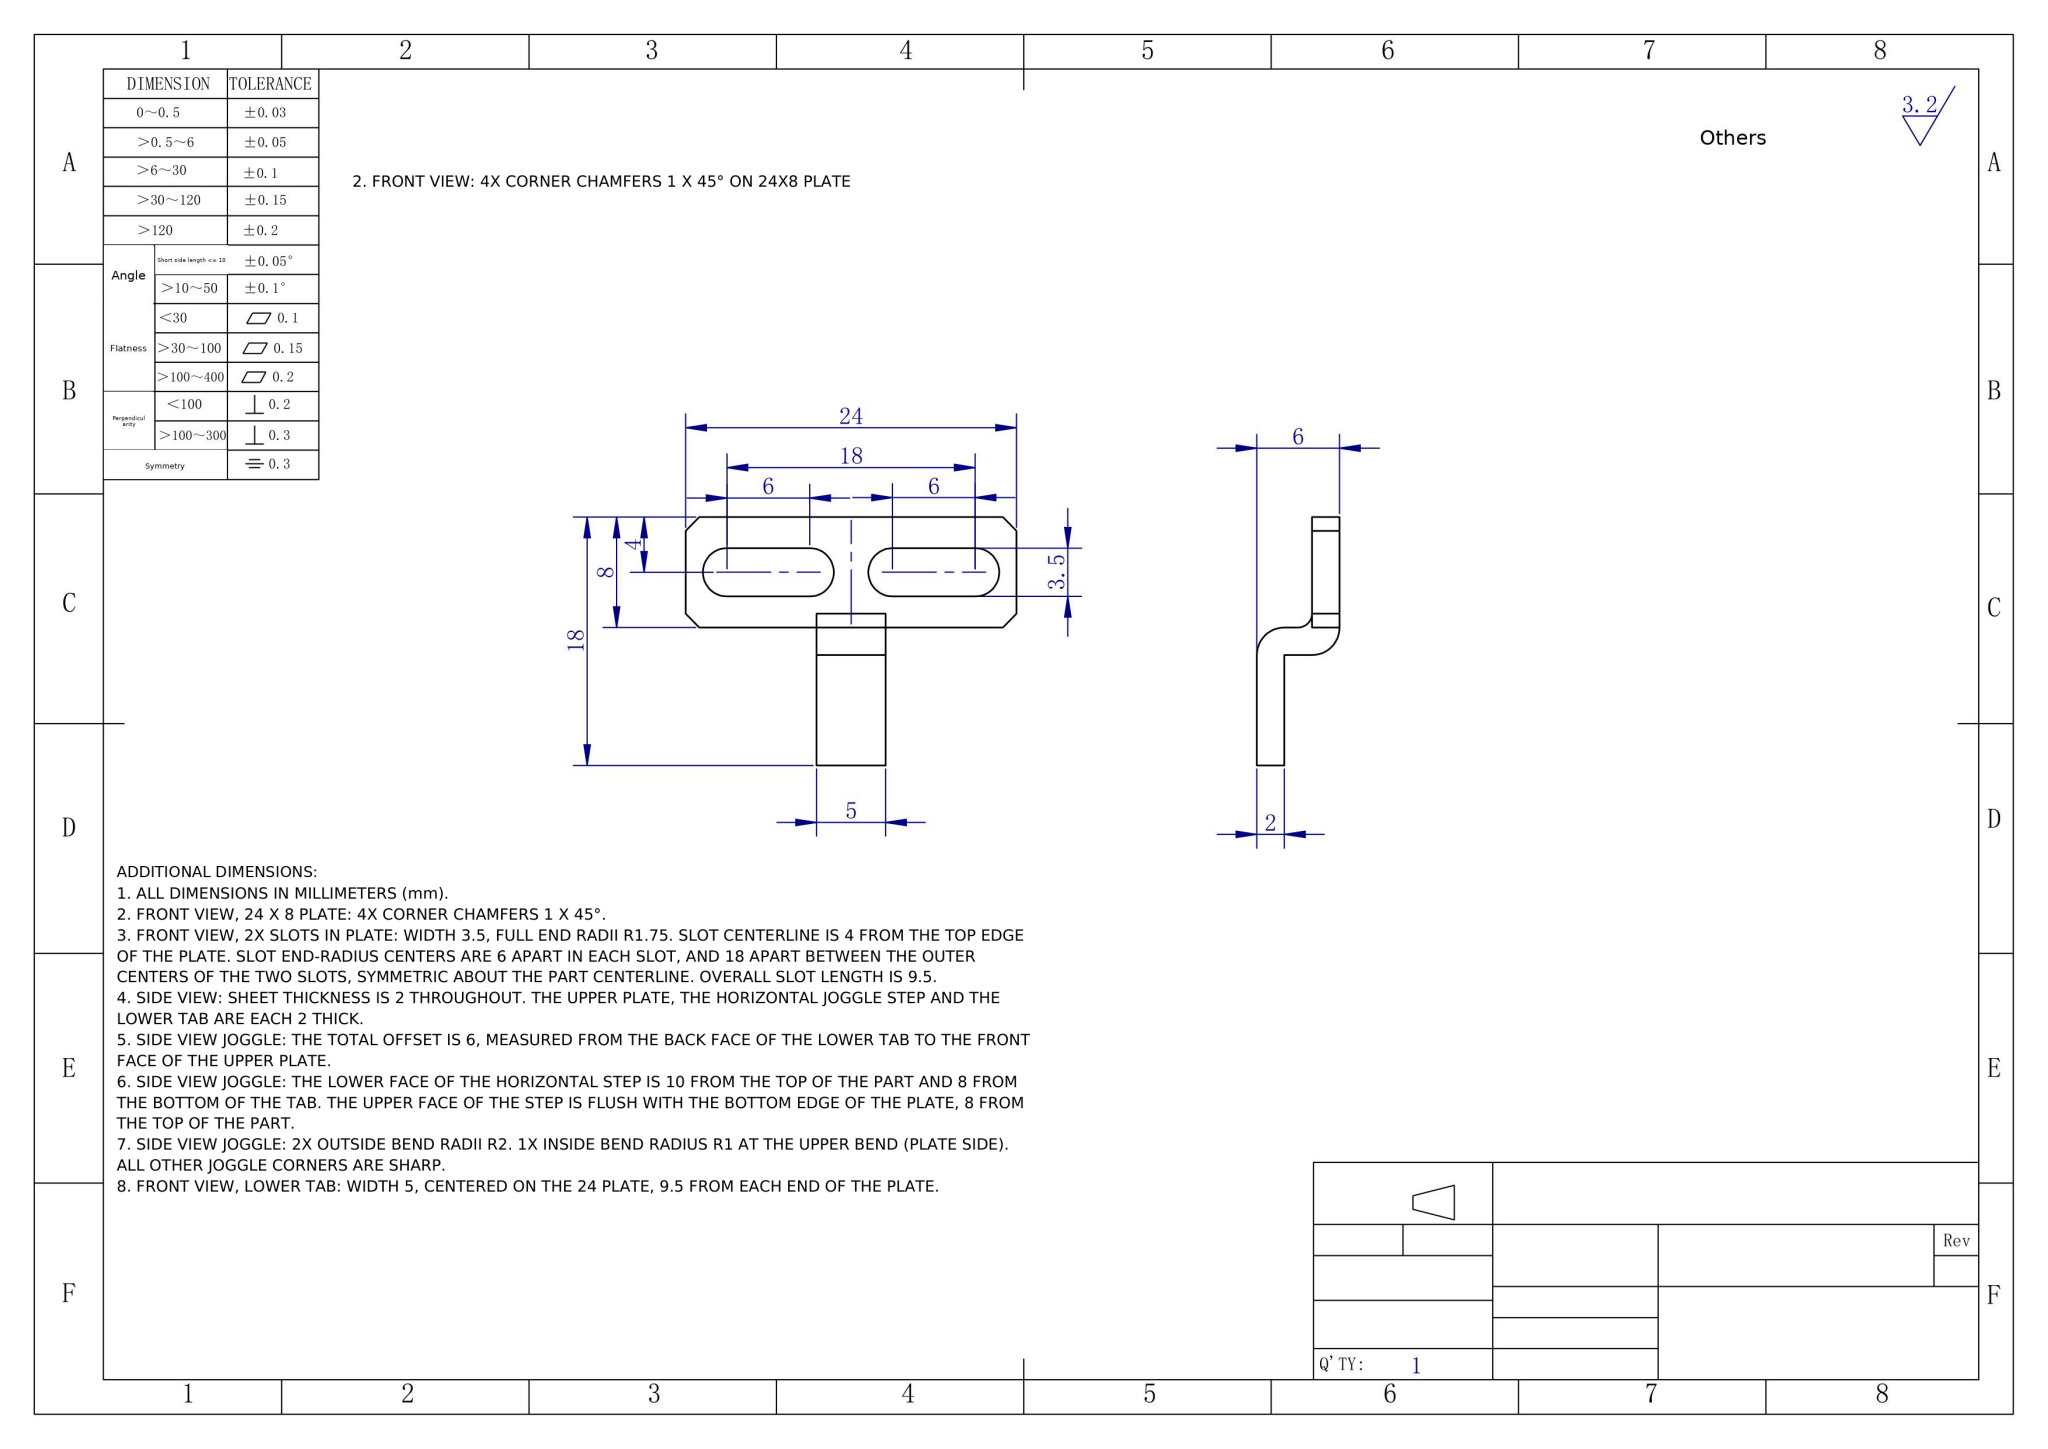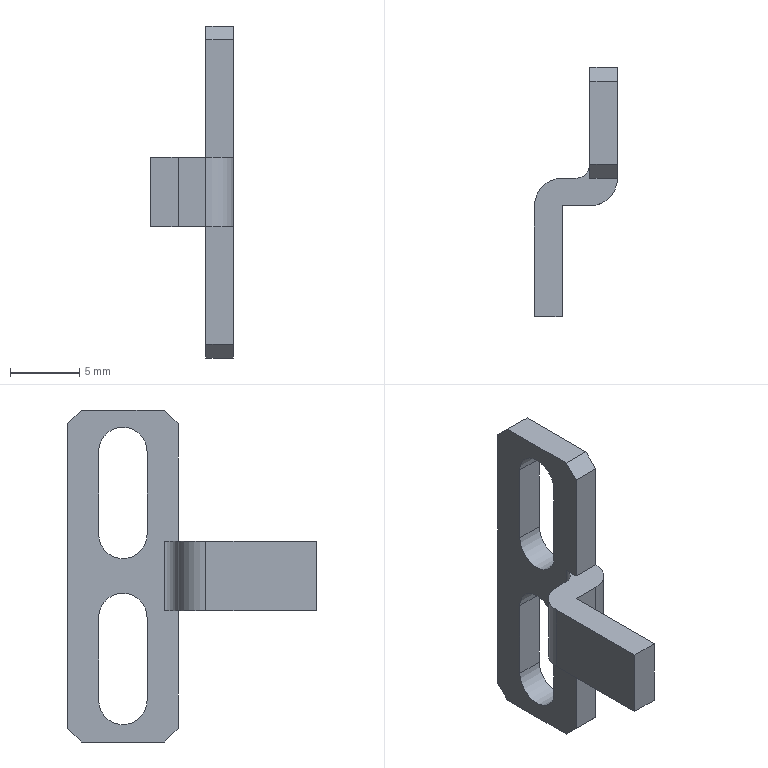Part | NX | mm | 1 solid | 31 faces | box 6 x 18 x 24 mm | volume 390 mm3 | plane 22 | cylinder 9 | commonest cylinder face diameters 3.5 x6 4 x2 2 x1
STEP:
#1=COLOUR_RGB('',0.7529,0.7529,0.7529);
#2=FILL_AREA_STYLE_COLOUR('',#1);
#3=FILL_AREA_STYLE('',(#2));
#4=SURFACE_STYLE_FILL_AREA(#3);
#5=SURFACE_SIDE_STYLE('',(#4));
#6=SURFACE_STYLE_USAGE(.BOTH.,#5);
#7=PRESENTATION_STYLE_ASSIGNMENT((#6));
#8=CARTESIAN_POINT('',(6.,4.,22.75));
#9=VERTEX_POINT('',#8);
#10=CARTESIAN_POINT('',(6.,5.75,21.));
#11=VERTEX_POINT('',#10);
#12=CARTESIAN_POINT('',(6.,4.,21.));
#13=DIRECTION('',(-1.,0.,0.));
#14=DIRECTION('',(0.,0.,1.));
#15=AXIS2_PLACEMENT_3D('',#12,#13,#14);
#16=CIRCLE('',#15,1.75);
#17=EDGE_CURVE('',#9,#11,#16,.T.);
#18=ORIENTED_EDGE('',*,*,#17,.F.);
#19=CARTESIAN_POINT('',(4.,4.,22.75));
#20=VERTEX_POINT('',#19);
#21=CARTESIAN_POINT('',(6.,4.,22.75));
#22=DIRECTION('',(-1.,0.,0.));
#23=VECTOR('',#22,1000.);
#24=LINE('',#21,#23);
#25=EDGE_CURVE('',#9,#20,#24,.T.);
#26=ORIENTED_EDGE('',*,*,#25,.T.);
#27=CARTESIAN_POINT('',(4.,5.75,21.));
#28=VERTEX_POINT('',#27);
#29=CARTESIAN_POINT('',(4.,4.,21.));
#30=DIRECTION('',(-1.,0.,0.));
#31=DIRECTION('',(0.,0.,1.));
#32=AXIS2_PLACEMENT_3D('',#29,#30,#31);
#33=CIRCLE('',#32,1.75);
#34=EDGE_CURVE('',#20,#28,#33,.T.);
#35=ORIENTED_EDGE('',*,*,#34,.T.);
#36=CARTESIAN_POINT('',(6.,5.75,21.));
#37=DIRECTION('',(-1.,0.,0.));
#38=VECTOR('',#37,1000.);
#39=LINE('',#36,#38);
#40=EDGE_CURVE('',#11,#28,#39,.T.);
#41=ORIENTED_EDGE('',*,*,#40,.F.);
#42=EDGE_LOOP('',(#18,#26,#35,#41));
#43=FACE_OUTER_BOUND('',#42,.T.);
#44=CARTESIAN_POINT('',(6.,4.,21.));
#45=DIRECTION('',(-1.,0.,0.));
#46=DIRECTION('',(0.,0.,1.));
#47=AXIS2_PLACEMENT_3D('',#44,#45,#46);
#48=CYLINDRICAL_SURFACE('',#47,1.75);
#49=ADVANCED_FACE('',(#43),#48,.F.);
#50=CARTESIAN_POINT('',(6.,4.,10.75));
#51=VERTEX_POINT('',#50);
#52=CARTESIAN_POINT('',(6.,5.75,9.));
#53=VERTEX_POINT('',#52);
#54=CARTESIAN_POINT('',(6.,4.,9.));
#55=DIRECTION('',(-1.,0.,0.));
#56=DIRECTION('',(0.,0.,1.));
#57=AXIS2_PLACEMENT_3D('',#54,#55,#56);
#58=CIRCLE('',#57,1.75);
#59=EDGE_CURVE('',#51,#53,#58,.T.);
#60=ORIENTED_EDGE('',*,*,#59,.F.);
#61=CARTESIAN_POINT('',(4.,4.,10.75));
#62=VERTEX_POINT('',#61);
#63=CARTESIAN_POINT('',(6.,4.,10.75));
#64=DIRECTION('',(-1.,0.,0.));
#65=VECTOR('',#64,1000.);
#66=LINE('',#63,#65);
#67=EDGE_CURVE('',#51,#62,#66,.T.);
#68=ORIENTED_EDGE('',*,*,#67,.T.);
#69=CARTESIAN_POINT('',(4.,5.75,9.));
#70=VERTEX_POINT('',#69);
#71=CARTESIAN_POINT('',(4.,4.,9.));
#72=DIRECTION('',(-1.,0.,0.));
#73=DIRECTION('',(0.,0.,1.));
#74=AXIS2_PLACEMENT_3D('',#71,#72,#73);
#75=CIRCLE('',#74,1.75);
#76=EDGE_CURVE('',#62,#70,#75,.T.);
#77=ORIENTED_EDGE('',*,*,#76,.T.);
#78=CARTESIAN_POINT('',(6.,5.75,9.));
#79=DIRECTION('',(-1.,0.,0.));
#80=VECTOR('',#79,1000.);
#81=LINE('',#78,#80);
#82=EDGE_CURVE('',#53,#70,#81,.T.);
#83=ORIENTED_EDGE('',*,*,#82,.F.);
#84=EDGE_LOOP('',(#60,#68,#77,#83));
#85=FACE_OUTER_BOUND('',#84,.T.);
#86=CARTESIAN_POINT('',(6.,4.,9.));
#87=DIRECTION('',(-1.,0.,0.));
#88=DIRECTION('',(0.,0.,1.));
#89=AXIS2_PLACEMENT_3D('',#86,#87,#88);
#90=CYLINDRICAL_SURFACE('',#89,1.75);
#91=ADVANCED_FACE('',(#85),#90,.F.);
#92=CARTESIAN_POINT('',(4.,1.,24.));
#93=VERTEX_POINT('',#92);
#94=CARTESIAN_POINT('',(4.,7.,24.));
#95=VERTEX_POINT('',#94);
#96=CARTESIAN_POINT('',(4.,0.,24.));
#97=DIRECTION('',(0.,1.,0.));
#98=VECTOR('',#97,1000.);
#99=LINE('',#96,#98);
#100=EDGE_CURVE('',#93,#95,#99,.T.);
#101=ORIENTED_EDGE('',*,*,#100,.F.);
#102=CARTESIAN_POINT('',(6.,1.,24.));
#103=VERTEX_POINT('',#102);
#104=CARTESIAN_POINT('',(0.,1.,24.));
#105=DIRECTION('',(1.,0.,0.));
#106=VECTOR('',#105,1000.);
#107=LINE('',#104,#106);
#108=EDGE_CURVE('',#93,#103,#107,.T.);
#109=ORIENTED_EDGE('',*,*,#108,.T.);
#110=CARTESIAN_POINT('',(6.,7.,24.));
#111=VERTEX_POINT('',#110);
#112=CARTESIAN_POINT('',(6.,0.,24.));
#113=DIRECTION('',(0.,1.,0.));
#114=VECTOR('',#113,1000.);
#115=LINE('',#112,#114);
#116=EDGE_CURVE('',#103,#111,#115,.T.);
#117=ORIENTED_EDGE('',*,*,#116,.T.);
#118=CARTESIAN_POINT('',(4.,7.,24.));
#119=DIRECTION('',(-1.,0.,0.));
#120=VECTOR('',#119,1000.);
#121=LINE('',#118,#120);
#122=EDGE_CURVE('',#111,#95,#121,.T.);
#123=ORIENTED_EDGE('',*,*,#122,.T.);
#124=EDGE_LOOP('',(#101,#109,#117,#123));
#125=FACE_OUTER_BOUND('',#124,.T.);
#126=CARTESIAN_POINT('',(0.,0.,24.));
#127=DIRECTION('',(0.,0.,-1.));
#128=DIRECTION('',(-1.,0.,0.));
#129=AXIS2_PLACEMENT_3D('',#126,#127,#128);
#130=PLANE('',#129);
#131=ADVANCED_FACE('',(#125),#130,.F.);
#132=CARTESIAN_POINT('',(6.,5.75,15.));
#133=VERTEX_POINT('',#132);
#134=CARTESIAN_POINT('',(6.,5.75,15.));
#135=DIRECTION('',(0.,-0.,-1.));
#136=VECTOR('',#135,1000.);
#137=LINE('',#134,#136);
#138=EDGE_CURVE('',#11,#133,#137,.T.);
#139=ORIENTED_EDGE('',*,*,#138,.T.);
#140=CARTESIAN_POINT('',(6.,2.25,15.));
#141=VERTEX_POINT('',#140);
#142=CARTESIAN_POINT('',(6.,4.,15.));
#143=DIRECTION('',(-1.,0.,0.));
#144=DIRECTION('',(0.,0.,1.));
#145=AXIS2_PLACEMENT_3D('',#142,#143,#144);
#146=CIRCLE('',#145,1.75);
#147=EDGE_CURVE('',#133,#141,#146,.T.);
#148=ORIENTED_EDGE('',*,*,#147,.T.);
#149=CARTESIAN_POINT('',(6.,2.25,21.));
#150=VERTEX_POINT('',#149);
#151=CARTESIAN_POINT('',(6.,2.25,15.));
#152=DIRECTION('',(0.,0.,1.));
#153=VECTOR('',#152,1000.);
#154=LINE('',#151,#153);
#155=EDGE_CURVE('',#141,#150,#154,.T.);
#156=ORIENTED_EDGE('',*,*,#155,.T.);
#157=CARTESIAN_POINT('',(6.,4.,21.));
#158=DIRECTION('',(-1.,0.,0.));
#159=DIRECTION('',(0.,0.,1.));
#160=AXIS2_PLACEMENT_3D('',#157,#158,#159);
#161=CIRCLE('',#160,1.75);
#162=EDGE_CURVE('',#150,#9,#161,.T.);
#163=ORIENTED_EDGE('',*,*,#162,.T.);
#164=ORIENTED_EDGE('',*,*,#17,.T.);
#165=EDGE_LOOP('',(#139,#148,#156,#163,#164));
#166=FACE_BOUND('',#165,.T.);
#167=CARTESIAN_POINT('',(6.,5.75,3.));
#168=VERTEX_POINT('',#167);
#169=CARTESIAN_POINT('',(6.,5.75,3.));
#170=DIRECTION('',(0.,-0.,-1.));
#171=VECTOR('',#170,1000.);
#172=LINE('',#169,#171);
#173=EDGE_CURVE('',#53,#168,#172,.T.);
#174=ORIENTED_EDGE('',*,*,#173,.T.);
#175=CARTESIAN_POINT('',(6.,2.25,3.));
#176=VERTEX_POINT('',#175);
#177=CARTESIAN_POINT('',(6.,4.,3.));
#178=DIRECTION('',(-1.,0.,0.));
#179=DIRECTION('',(0.,0.,1.));
#180=AXIS2_PLACEMENT_3D('',#177,#178,#179);
#181=CIRCLE('',#180,1.75);
#182=EDGE_CURVE('',#168,#176,#181,.T.);
#183=ORIENTED_EDGE('',*,*,#182,.T.);
#184=CARTESIAN_POINT('',(6.,2.25,9.));
#185=VERTEX_POINT('',#184);
#186=CARTESIAN_POINT('',(6.,2.25,3.));
#187=DIRECTION('',(0.,0.,1.));
#188=VECTOR('',#187,1000.);
#189=LINE('',#186,#188);
#190=EDGE_CURVE('',#176,#185,#189,.T.);
#191=ORIENTED_EDGE('',*,*,#190,.T.);
#192=CARTESIAN_POINT('',(6.,4.,9.));
#193=DIRECTION('',(-1.,0.,0.));
#194=DIRECTION('',(0.,0.,1.));
#195=AXIS2_PLACEMENT_3D('',#192,#193,#194);
#196=CIRCLE('',#195,1.75);
#197=EDGE_CURVE('',#185,#51,#196,.T.);
#198=ORIENTED_EDGE('',*,*,#197,.T.);
#199=ORIENTED_EDGE('',*,*,#59,.T.);
#200=EDGE_LOOP('',(#174,#183,#191,#198,#199));
#201=FACE_BOUND('',#200,.T.);
#202=ORIENTED_EDGE('',*,*,#116,.F.);
#203=CARTESIAN_POINT('',(6.,0.,23.));
#204=VERTEX_POINT('',#203);
#205=CARTESIAN_POINT('',(6.,1.,24.));
#206=DIRECTION('',(0.,-0.7071,-0.7071));
#207=VECTOR('',#206,1000.);
#208=LINE('',#205,#207);
#209=EDGE_CURVE('',#103,#204,#208,.T.);
#210=ORIENTED_EDGE('',*,*,#209,.T.);
#211=CARTESIAN_POINT('',(6.,0.,14.5));
#212=VERTEX_POINT('',#211);
#213=CARTESIAN_POINT('',(6.,0.,24.));
#214=DIRECTION('',(0.,0.,-1.));
#215=VECTOR('',#214,1000.);
#216=LINE('',#213,#215);
#217=EDGE_CURVE('',#204,#212,#216,.T.);
#218=ORIENTED_EDGE('',*,*,#217,.T.);
#219=CARTESIAN_POINT('',(6.,0.,9.5));
#220=VERTEX_POINT('',#219);
#221=CARTESIAN_POINT('',(6.,0.,24.));
#222=DIRECTION('',(0.,0.,-1.));
#223=VECTOR('',#222,1000.);
#224=LINE('',#221,#223);
#225=EDGE_CURVE('',#212,#220,#224,.T.);
#226=ORIENTED_EDGE('',*,*,#225,.T.);
#227=CARTESIAN_POINT('',(6.,-0.,1.));
#228=VERTEX_POINT('',#227);
#229=CARTESIAN_POINT('',(6.,0.,24.));
#230=DIRECTION('',(0.,0.,-1.));
#231=VECTOR('',#230,1000.);
#232=LINE('',#229,#231);
#233=EDGE_CURVE('',#220,#228,#232,.T.);
#234=ORIENTED_EDGE('',*,*,#233,.T.);
#235=CARTESIAN_POINT('',(6.,1.,0.));
#236=VERTEX_POINT('',#235);
#237=CARTESIAN_POINT('',(6.,0.,1.));
#238=DIRECTION('',(0.,0.7071,-0.7071));
#239=VECTOR('',#238,1000.);
#240=LINE('',#237,#239);
#241=EDGE_CURVE('',#228,#236,#240,.T.);
#242=ORIENTED_EDGE('',*,*,#241,.T.);
#243=CARTESIAN_POINT('',(6.,7.,0.));
#244=VERTEX_POINT('',#243);
#245=CARTESIAN_POINT('',(6.,0.,0.));
#246=DIRECTION('',(0.,1.,0.));
#247=VECTOR('',#246,1000.);
#248=LINE('',#245,#247);
#249=EDGE_CURVE('',#236,#244,#248,.T.);
#250=ORIENTED_EDGE('',*,*,#249,.T.);
#251=CARTESIAN_POINT('',(6.,8.,1.));
#252=VERTEX_POINT('',#251);
#253=CARTESIAN_POINT('',(6.,7.,0.));
#254=DIRECTION('',(0.,0.7071,0.7071));
#255=VECTOR('',#254,1000.);
#256=LINE('',#253,#255);
#257=EDGE_CURVE('',#244,#252,#256,.T.);
#258=ORIENTED_EDGE('',*,*,#257,.T.);
#259=CARTESIAN_POINT('',(6.,8.,23.));
#260=VERTEX_POINT('',#259);
#261=CARTESIAN_POINT('',(6.,8.,24.));
#262=DIRECTION('',(0.,0.,-1.));
#263=VECTOR('',#262,1000.);
#264=LINE('',#261,#263);
#265=EDGE_CURVE('',#260,#252,#264,.T.);
#266=ORIENTED_EDGE('',*,*,#265,.F.);
#267=CARTESIAN_POINT('',(6.,8.,23.));
#268=DIRECTION('',(0.,-0.7071,0.7071));
#269=VECTOR('',#268,1000.);
#270=LINE('',#267,#269);
#271=EDGE_CURVE('',#260,#111,#270,.T.);
#272=ORIENTED_EDGE('',*,*,#271,.T.);
#273=EDGE_LOOP('',(#202,#210,#218,#226,#234,#242,#250,#258,#266,#272));
#274=FACE_OUTER_BOUND('',#273,.T.);
#275=CARTESIAN_POINT('',(6.,0.,24.));
#276=DIRECTION('',(-1.,0.,0.));
#277=DIRECTION('',(0.,0.,1.));
#278=AXIS2_PLACEMENT_3D('',#275,#276,#277);
#279=PLANE('',#278);
#280=ADVANCED_FACE('',(#166,#201,#274),#279,.F.);
#281=CARTESIAN_POINT('',(4.,8.,23.));
#282=VERTEX_POINT('',#281);
#283=CARTESIAN_POINT('',(4.,8.,1.));
#284=VERTEX_POINT('',#283);
#285=CARTESIAN_POINT('',(4.,8.,24.));
#286=DIRECTION('',(0.,0.,-1.));
#287=VECTOR('',#286,1000.);
#288=LINE('',#285,#287);
#289=EDGE_CURVE('',#282,#284,#288,.T.);
#290=ORIENTED_EDGE('',*,*,#289,.F.);
#291=CARTESIAN_POINT('',(6.,8.,23.));
#292=DIRECTION('',(1.,0.,0.));
#293=VECTOR('',#292,1000.);
#294=LINE('',#291,#293);
#295=EDGE_CURVE('',#282,#260,#294,.T.);
#296=ORIENTED_EDGE('',*,*,#295,.T.);
#297=ORIENTED_EDGE('',*,*,#265,.T.);
#298=CARTESIAN_POINT('',(4.,8.,1.));
#299=DIRECTION('',(-1.,0.,0.));
#300=VECTOR('',#299,1000.);
#301=LINE('',#298,#300);
#302=EDGE_CURVE('',#252,#284,#301,.T.);
#303=ORIENTED_EDGE('',*,*,#302,.T.);
#304=EDGE_LOOP('',(#290,#296,#297,#303));
#305=FACE_OUTER_BOUND('',#304,.T.);
#306=CARTESIAN_POINT('',(4.,8.,24.));
#307=DIRECTION('',(0.,1.,0.));
#308=DIRECTION('',(0.,0.,1.));
#309=AXIS2_PLACEMENT_3D('',#306,#307,#308);
#310=PLANE('',#309);
#311=ADVANCED_FACE('',(#305),#310,.T.);
#312=CARTESIAN_POINT('',(4.,5.75,15.));
#313=VERTEX_POINT('',#312);
#314=CARTESIAN_POINT('',(4.,2.25,15.));
#315=VERTEX_POINT('',#314);
#316=CARTESIAN_POINT('',(4.,4.,15.));
#317=DIRECTION('',(-1.,0.,0.));
#318=DIRECTION('',(0.,0.,1.));
#319=AXIS2_PLACEMENT_3D('',#316,#317,#318);
#320=CIRCLE('',#319,1.75);
#321=EDGE_CURVE('',#313,#315,#320,.T.);
#322=ORIENTED_EDGE('',*,*,#321,.F.);
#323=CARTESIAN_POINT('',(4.,5.75,15.));
#324=DIRECTION('',(0.,-0.,-1.));
#325=VECTOR('',#324,1000.);
#326=LINE('',#323,#325);
#327=EDGE_CURVE('',#28,#313,#326,.T.);
#328=ORIENTED_EDGE('',*,*,#327,.F.);
#329=ORIENTED_EDGE('',*,*,#34,.F.);
#330=CARTESIAN_POINT('',(4.,2.25,21.));
#331=VERTEX_POINT('',#330);
#332=CARTESIAN_POINT('',(4.,4.,21.));
#333=DIRECTION('',(-1.,0.,0.));
#334=DIRECTION('',(0.,0.,1.));
#335=AXIS2_PLACEMENT_3D('',#332,#333,#334);
#336=CIRCLE('',#335,1.75);
#337=EDGE_CURVE('',#331,#20,#336,.T.);
#338=ORIENTED_EDGE('',*,*,#337,.F.);
#339=CARTESIAN_POINT('',(4.,2.25,15.));
#340=DIRECTION('',(0.,0.,1.));
#341=VECTOR('',#340,1000.);
#342=LINE('',#339,#341);
#343=EDGE_CURVE('',#315,#331,#342,.T.);
#344=ORIENTED_EDGE('',*,*,#343,.F.);
#345=EDGE_LOOP('',(#322,#328,#329,#338,#344));
#346=FACE_BOUND('',#345,.T.);
#347=CARTESIAN_POINT('',(4.,5.75,3.));
#348=VERTEX_POINT('',#347);
#349=CARTESIAN_POINT('',(4.,2.25,3.));
#350=VERTEX_POINT('',#349);
#351=CARTESIAN_POINT('',(4.,4.,3.));
#352=DIRECTION('',(-1.,0.,0.));
#353=DIRECTION('',(0.,0.,1.));
#354=AXIS2_PLACEMENT_3D('',#351,#352,#353);
#355=CIRCLE('',#354,1.75);
#356=EDGE_CURVE('',#348,#350,#355,.T.);
#357=ORIENTED_EDGE('',*,*,#356,.F.);
#358=CARTESIAN_POINT('',(4.,5.75,3.));
#359=DIRECTION('',(0.,-0.,-1.));
#360=VECTOR('',#359,1000.);
#361=LINE('',#358,#360);
#362=EDGE_CURVE('',#70,#348,#361,.T.);
#363=ORIENTED_EDGE('',*,*,#362,.F.);
#364=ORIENTED_EDGE('',*,*,#76,.F.);
#365=CARTESIAN_POINT('',(4.,2.25,9.));
#366=VERTEX_POINT('',#365);
#367=CARTESIAN_POINT('',(4.,4.,9.));
#368=DIRECTION('',(-1.,0.,0.));
#369=DIRECTION('',(0.,0.,1.));
#370=AXIS2_PLACEMENT_3D('',#367,#368,#369);
#371=CIRCLE('',#370,1.75);
#372=EDGE_CURVE('',#366,#62,#371,.T.);
#373=ORIENTED_EDGE('',*,*,#372,.F.);
#374=CARTESIAN_POINT('',(4.,2.25,3.));
#375=DIRECTION('',(0.,0.,1.));
#376=VECTOR('',#375,1000.);
#377=LINE('',#374,#376);
#378=EDGE_CURVE('',#350,#366,#377,.T.);
#379=ORIENTED_EDGE('',*,*,#378,.F.);
#380=EDGE_LOOP('',(#357,#363,#364,#373,#379));
#381=FACE_BOUND('',#380,.T.);
#382=CARTESIAN_POINT('',(4.,0.,23.));
#383=VERTEX_POINT('',#382);
#384=CARTESIAN_POINT('',(4.,0.,14.5));
#385=VERTEX_POINT('',#384);
#386=CARTESIAN_POINT('',(4.,0.,24.));
#387=DIRECTION('',(0.,0.,-1.));
#388=VECTOR('',#387,1000.);
#389=LINE('',#386,#388);
#390=EDGE_CURVE('',#383,#385,#389,.T.);
#391=ORIENTED_EDGE('',*,*,#390,.F.);
#392=CARTESIAN_POINT('',(4.,0.5,23.5));
#393=DIRECTION('',(0.,0.7071,0.7071));
#394=VECTOR('',#393,1000.);
#395=LINE('',#392,#394);
#396=EDGE_CURVE('',#383,#93,#395,.T.);
#397=ORIENTED_EDGE('',*,*,#396,.T.);
#398=ORIENTED_EDGE('',*,*,#100,.T.);
#399=CARTESIAN_POINT('',(4.,3.5,27.5));
#400=DIRECTION('',(0.,0.7071,-0.7071));
#401=VECTOR('',#400,1000.);
#402=LINE('',#399,#401);
#403=EDGE_CURVE('',#95,#282,#402,.T.);
#404=ORIENTED_EDGE('',*,*,#403,.T.);
#405=ORIENTED_EDGE('',*,*,#289,.T.);
#406=CARTESIAN_POINT('',(4.,7.,0.));
#407=VERTEX_POINT('',#406);
#408=CARTESIAN_POINT('',(4.,15.5,8.5));
#409=DIRECTION('',(0.,-0.7071,-0.7071));
#410=VECTOR('',#409,1000.);
#411=LINE('',#408,#410);
#412=EDGE_CURVE('',#284,#407,#411,.T.);
#413=ORIENTED_EDGE('',*,*,#412,.T.);
#414=CARTESIAN_POINT('',(4.,1.,0.));
#415=VERTEX_POINT('',#414);
#416=CARTESIAN_POINT('',(4.,0.,0.));
#417=DIRECTION('',(0.,1.,0.));
#418=VECTOR('',#417,1000.);
#419=LINE('',#416,#418);
#420=EDGE_CURVE('',#415,#407,#419,.T.);
#421=ORIENTED_EDGE('',*,*,#420,.F.);
#422=CARTESIAN_POINT('',(4.,-0.,1.));
#423=VERTEX_POINT('',#422);
#424=CARTESIAN_POINT('',(4.,-11.5,12.5));
#425=DIRECTION('',(0.,-0.7071,0.7071));
#426=VECTOR('',#425,1000.);
#427=LINE('',#424,#426);
#428=EDGE_CURVE('',#415,#423,#427,.T.);
#429=ORIENTED_EDGE('',*,*,#428,.T.);
#430=CARTESIAN_POINT('',(4.,0.,9.5));
#431=VERTEX_POINT('',#430);
#432=CARTESIAN_POINT('',(4.,0.,24.));
#433=DIRECTION('',(0.,0.,-1.));
#434=VECTOR('',#433,1000.);
#435=LINE('',#432,#434);
#436=EDGE_CURVE('',#431,#423,#435,.T.);
#437=ORIENTED_EDGE('',*,*,#436,.F.);
#438=CARTESIAN_POINT('',(4.,1.,9.5));
#439=VERTEX_POINT('',#438);
#440=CARTESIAN_POINT('',(4.,0.,9.5));
#441=DIRECTION('',(0.,1.,0.));
#442=VECTOR('',#441,1000.);
#443=LINE('',#440,#442);
#444=EDGE_CURVE('',#431,#439,#443,.T.);
#445=ORIENTED_EDGE('',*,*,#444,.T.);
#446=CARTESIAN_POINT('',(4.,1.,14.5));
#447=VERTEX_POINT('',#446);
#448=CARTESIAN_POINT('',(4.,1.,14.5));
#449=DIRECTION('',(0.,0.,1.));
#450=VECTOR('',#449,1000.);
#451=LINE('',#448,#450);
#452=EDGE_CURVE('',#439,#447,#451,.T.);
#453=ORIENTED_EDGE('',*,*,#452,.T.);
#454=CARTESIAN_POINT('',(4.,0.,14.5));
#455=DIRECTION('',(0.,-1.,0.));
#456=VECTOR('',#455,1000.);
#457=LINE('',#454,#456);
#458=EDGE_CURVE('',#447,#385,#457,.T.);
#459=ORIENTED_EDGE('',*,*,#458,.T.);
#460=EDGE_LOOP('',(#391,#397,#398,#404,#405,#413,#421,#429,#437,#445,#453,#459));
#461=FACE_OUTER_BOUND('',#460,.T.);
#462=CARTESIAN_POINT('',(4.,0.,24.));
#463=DIRECTION('',(-1.,0.,0.));
#464=DIRECTION('',(0.,0.,1.));
#465=AXIS2_PLACEMENT_3D('',#462,#463,#464);
#466=PLANE('',#465);
#467=ADVANCED_FACE('',(#346,#381,#461),#466,.T.);
#468=CARTESIAN_POINT('',(3.,0.,14.5));
#469=VERTEX_POINT('',#468);
#470=CARTESIAN_POINT('',(2.,0.,14.5));
#471=VERTEX_POINT('',#470);
#472=CARTESIAN_POINT('',(0.,0.,14.5));
#473=DIRECTION('',(-1.,0.,0.));
#474=VECTOR('',#473,1000.);
#475=LINE('',#472,#474);
#476=EDGE_CURVE('',#469,#471,#475,.T.);
#477=ORIENTED_EDGE('',*,*,#476,.F.);
#478=CARTESIAN_POINT('',(3.,0.,9.5));
#479=VERTEX_POINT('',#478);
#480=CARTESIAN_POINT('',(3.,0.,9.5));
#481=DIRECTION('',(0.,0.,-1.));
#482=VECTOR('',#481,1000.);
#483=LINE('',#480,#482);
#484=EDGE_CURVE('',#469,#479,#483,.T.);
#485=ORIENTED_EDGE('',*,*,#484,.T.);
#486=CARTESIAN_POINT('',(2.,0.,9.5));
#487=VERTEX_POINT('',#486);
#488=CARTESIAN_POINT('',(0.,0.,9.5));
#489=DIRECTION('',(1.,0.,0.));
#490=VECTOR('',#489,1000.);
#491=LINE('',#488,#490);
#492=EDGE_CURVE('',#487,#479,#491,.T.);
#493=ORIENTED_EDGE('',*,*,#492,.F.);
#494=CARTESIAN_POINT('',(2.,0.,24.));
#495=DIRECTION('',(0.,0.,1.));
#496=VECTOR('',#495,1000.);
#497=LINE('',#494,#496);
#498=EDGE_CURVE('',#487,#471,#497,.T.);
#499=ORIENTED_EDGE('',*,*,#498,.T.);
#500=EDGE_LOOP('',(#477,#485,#493,#499));
#501=FACE_OUTER_BOUND('',#500,.T.);
#502=CARTESIAN_POINT('',(0.,0.,24.));
#503=DIRECTION('',(0.,1.,0.));
#504=DIRECTION('',(0.,0.,1.));
#505=AXIS2_PLACEMENT_3D('',#502,#503,#504);
#506=PLANE('',#505);
#507=ADVANCED_FACE('',(#501),#506,.T.);
#508=CARTESIAN_POINT('',(0.,-2.,14.5));
#509=VERTEX_POINT('',#508);
#510=CARTESIAN_POINT('',(0.,-10.,14.5));
#511=VERTEX_POINT('',#510);
#512=CARTESIAN_POINT('',(0.,-10.,14.5));
#513=DIRECTION('',(0.,-1.,0.));
#514=VECTOR('',#513,1000.);
#515=LINE('',#512,#514);
#516=EDGE_CURVE('',#509,#511,#515,.T.);
#517=ORIENTED_EDGE('',*,*,#516,.F.);
#518=CARTESIAN_POINT('',(0.,-2.,9.5));
#519=VERTEX_POINT('',#518);
#520=CARTESIAN_POINT('',(0.,-2.,24.));
#521=DIRECTION('',(0.,0.,-1.));
#522=VECTOR('',#521,1000.);
#523=LINE('',#520,#522);
#524=EDGE_CURVE('',#509,#519,#523,.T.);
#525=ORIENTED_EDGE('',*,*,#524,.T.);
#526=CARTESIAN_POINT('',(0.,-10.,9.5));
#527=VERTEX_POINT('',#526);
#528=CARTESIAN_POINT('',(0.,-10.,9.5));
#529=DIRECTION('',(0.,1.,0.));
#530=VECTOR('',#529,1000.);
#531=LINE('',#528,#530);
#532=EDGE_CURVE('',#527,#519,#531,.T.);
#533=ORIENTED_EDGE('',*,*,#532,.F.);
#534=CARTESIAN_POINT('',(0.,-10.,24.));
#535=DIRECTION('',(0.,0.,-1.));
#536=VECTOR('',#535,1000.);
#537=LINE('',#534,#536);
#538=EDGE_CURVE('',#511,#527,#537,.T.);
#539=ORIENTED_EDGE('',*,*,#538,.F.);
#540=EDGE_LOOP('',(#517,#525,#533,#539));
#541=FACE_OUTER_BOUND('',#540,.T.);
#542=CARTESIAN_POINT('',(0.,-10.,24.));
#543=DIRECTION('',(-1.,0.,0.));
#544=DIRECTION('',(0.,0.,1.));
#545=AXIS2_PLACEMENT_3D('',#542,#543,#544);
#546=PLANE('',#545);
#547=ADVANCED_FACE('',(#541),#546,.T.);
#548=CARTESIAN_POINT('',(2.,-10.,14.5));
#549=VERTEX_POINT('',#548);
#550=CARTESIAN_POINT('',(3.,-10.,14.5));
#551=DIRECTION('',(-1.,0.,0.));
#552=VECTOR('',#551,1000.);
#553=LINE('',#550,#552);
#554=EDGE_CURVE('',#549,#511,#553,.T.);
#555=ORIENTED_EDGE('',*,*,#554,.T.);
#556=ORIENTED_EDGE('',*,*,#538,.T.);
#557=CARTESIAN_POINT('',(2.,-10.,9.5));
#558=VERTEX_POINT('',#557);
#559=CARTESIAN_POINT('',(3.,-10.,9.5));
#560=DIRECTION('',(-1.,0.,0.));
#561=VECTOR('',#560,1000.);
#562=LINE('',#559,#561);
#563=EDGE_CURVE('',#558,#527,#562,.T.);
#564=ORIENTED_EDGE('',*,*,#563,.F.);
#565=CARTESIAN_POINT('',(2.,-10.,24.));
#566=DIRECTION('',(0.,0.,-1.));
#567=VECTOR('',#566,1000.);
#568=LINE('',#565,#567);
#569=EDGE_CURVE('',#549,#558,#568,.T.);
#570=ORIENTED_EDGE('',*,*,#569,.F.);
#571=EDGE_LOOP('',(#555,#556,#564,#570));
#572=FACE_OUTER_BOUND('',#571,.T.);
#573=CARTESIAN_POINT('',(2.,-10.,24.));
#574=DIRECTION('',(0.,-1.,0.));
#575=DIRECTION('',(0.,0.,-1.));
#576=AXIS2_PLACEMENT_3D('',#573,#574,#575);
#577=PLANE('',#576);
#578=ADVANCED_FACE('',(#572),#577,.T.);
#579=CARTESIAN_POINT('',(2.,-2.,14.5));
#580=VERTEX_POINT('',#579);
#581=CARTESIAN_POINT('',(2.,-2.,9.5));
#582=VERTEX_POINT('',#581);
#583=CARTESIAN_POINT('',(2.,-2.,24.));
#584=DIRECTION('',(0.,0.,-1.));
#585=VECTOR('',#584,1000.);
#586=LINE('',#583,#585);
#587=EDGE_CURVE('',#580,#582,#586,.T.);
#588=ORIENTED_EDGE('',*,*,#587,.F.);
#589=CARTESIAN_POINT('',(2.,-10.,14.5));
#590=DIRECTION('',(0.,-1.,0.));
#591=VECTOR('',#590,1000.);
#592=LINE('',#589,#591);
#593=EDGE_CURVE('',#580,#549,#592,.T.);
#594=ORIENTED_EDGE('',*,*,#593,.T.);
#595=ORIENTED_EDGE('',*,*,#569,.T.);
#596=CARTESIAN_POINT('',(2.,-10.,9.5));
#597=DIRECTION('',(0.,1.,0.));
#598=VECTOR('',#597,1000.);
#599=LINE('',#596,#598);
#600=EDGE_CURVE('',#558,#582,#599,.T.);
#601=ORIENTED_EDGE('',*,*,#600,.T.);
#602=EDGE_LOOP('',(#588,#594,#595,#601));
#603=FACE_OUTER_BOUND('',#602,.T.);
#604=CARTESIAN_POINT('',(2.,-10.,24.));
#605=DIRECTION('',(-1.,0.,0.));
#606=DIRECTION('',(0.,0.,1.));
#607=AXIS2_PLACEMENT_3D('',#604,#605,#606);
#608=PLANE('',#607);
#609=ADVANCED_FACE('',(#603),#608,.F.);
#610=CARTESIAN_POINT('',(4.,-2.,9.5));
#611=VERTEX_POINT('',#610);
#612=CARTESIAN_POINT('',(4.,-2.,14.5));
#613=VERTEX_POINT('',#612);
#614=CARTESIAN_POINT('',(4.,-2.,24.));
#615=DIRECTION('',(0.,0.,1.));
#616=VECTOR('',#615,1000.);
#617=LINE('',#614,#616);
#618=EDGE_CURVE('',#611,#613,#617,.T.);
#619=ORIENTED_EDGE('',*,*,#618,.T.);
#620=CARTESIAN_POINT('',(0.,-2.,14.5));
#621=DIRECTION('',(-1.,0.,0.));
#622=VECTOR('',#621,1000.);
#623=LINE('',#620,#622);
#624=EDGE_CURVE('',#613,#580,#623,.T.);
#625=ORIENTED_EDGE('',*,*,#624,.T.);
#626=ORIENTED_EDGE('',*,*,#587,.T.);
#627=CARTESIAN_POINT('',(0.,-2.,9.5));
#628=DIRECTION('',(1.,0.,0.));
#629=VECTOR('',#628,1000.);
#630=LINE('',#627,#629);
#631=EDGE_CURVE('',#582,#611,#630,.T.);
#632=ORIENTED_EDGE('',*,*,#631,.T.);
#633=EDGE_LOOP('',(#619,#625,#626,#632));
#634=FACE_OUTER_BOUND('',#633,.T.);
#635=CARTESIAN_POINT('',(0.,-2.,24.));
#636=DIRECTION('',(0.,1.,0.));
#637=DIRECTION('',(0.,0.,1.));
#638=AXIS2_PLACEMENT_3D('',#635,#636,#637);
#639=PLANE('',#638);
#640=ADVANCED_FACE('',(#634),#639,.F.);
#641=ORIENTED_EDGE('',*,*,#249,.F.);
#642=CARTESIAN_POINT('',(4.,1.,0.));
#643=DIRECTION('',(-1.,0.,0.));
#644=VECTOR('',#643,1000.);
#645=LINE('',#642,#644);
#646=EDGE_CURVE('',#236,#415,#645,.T.);
#647=ORIENTED_EDGE('',*,*,#646,.T.);
#648=ORIENTED_EDGE('',*,*,#420,.T.);
#649=CARTESIAN_POINT('',(0.,7.,0.));
#650=DIRECTION('',(1.,0.,0.));
#651=VECTOR('',#650,1000.);
#652=LINE('',#649,#651);
#653=EDGE_CURVE('',#407,#244,#652,.T.);
#654=ORIENTED_EDGE('',*,*,#653,.T.);
#655=EDGE_LOOP('',(#641,#647,#648,#654));
#656=FACE_OUTER_BOUND('',#655,.T.);
#657=CARTESIAN_POINT('',(0.,0.,0.));
#658=DIRECTION('',(0.,0.,-1.));
#659=DIRECTION('',(-1.,0.,0.));
#660=AXIS2_PLACEMENT_3D('',#657,#658,#659);
#661=PLANE('',#660);
#662=ADVANCED_FACE('',(#656),#661,.T.);
#663=CARTESIAN_POINT('',(4.,0.,14.5));
#664=DIRECTION('',(0.,0.,1.));
#665=DIRECTION('',(0.,1.,0.));
#666=AXIS2_PLACEMENT_3D('',#663,#664,#665);
#667=CIRCLE('',#666,2.);
#668=EDGE_CURVE('',#613,#212,#667,.T.);
#669=ORIENTED_EDGE('',*,*,#668,.F.);
#670=ORIENTED_EDGE('',*,*,#618,.F.);
#671=CARTESIAN_POINT('',(4.,0.,9.5));
#672=DIRECTION('',(0.,0.,-1.));
#673=DIRECTION('',(1.,0.,0.));
#674=AXIS2_PLACEMENT_3D('',#671,#672,#673);
#675=CIRCLE('',#674,2.);
#676=EDGE_CURVE('',#220,#611,#675,.T.);
#677=ORIENTED_EDGE('',*,*,#676,.F.);
#678=ORIENTED_EDGE('',*,*,#225,.F.);
#679=EDGE_LOOP('',(#669,#670,#677,#678));
#680=FACE_OUTER_BOUND('',#679,.T.);
#681=CARTESIAN_POINT('',(4.,0.,24.));
#682=DIRECTION('',(0.,0.,-1.));
#683=DIRECTION('',(-1.,0.,0.));
#684=AXIS2_PLACEMENT_3D('',#681,#682,#683);
#685=CYLINDRICAL_SURFACE('',#684,2.);
#686=ADVANCED_FACE('',(#680),#685,.T.);
#687=CARTESIAN_POINT('',(2.,-2.,14.5));
#688=DIRECTION('',(0.,0.,1.));
#689=DIRECTION('',(-1.,0.,0.));
#690=AXIS2_PLACEMENT_3D('',#687,#688,#689);
#691=CIRCLE('',#690,2.);
#692=EDGE_CURVE('',#471,#509,#691,.T.);
#693=ORIENTED_EDGE('',*,*,#692,.F.);
#694=ORIENTED_EDGE('',*,*,#498,.F.);
#695=CARTESIAN_POINT('',(2.,-2.,9.5));
#696=DIRECTION('',(0.,0.,-1.));
#697=DIRECTION('',(1.,0.,0.));
#698=AXIS2_PLACEMENT_3D('',#695,#696,#697);
#699=CIRCLE('',#698,2.);
#700=EDGE_CURVE('',#519,#487,#699,.T.);
#701=ORIENTED_EDGE('',*,*,#700,.F.);
#702=ORIENTED_EDGE('',*,*,#524,.F.);
#703=EDGE_LOOP('',(#693,#694,#701,#702));
#704=FACE_OUTER_BOUND('',#703,.T.);
#705=CARTESIAN_POINT('',(2.,-2.,24.));
#706=DIRECTION('',(0.,0.,-1.));
#707=DIRECTION('',(-1.,0.,0.));
#708=AXIS2_PLACEMENT_3D('',#705,#706,#707);
#709=CYLINDRICAL_SURFACE('',#708,2.);
#710=ADVANCED_FACE('',(#704),#709,.T.);
#711=ORIENTED_EDGE('',*,*,#356,.T.);
#712=CARTESIAN_POINT('',(6.,2.25,3.));
#713=DIRECTION('',(-1.,0.,0.));
#714=VECTOR('',#713,1000.);
#715=LINE('',#712,#714);
#716=EDGE_CURVE('',#176,#350,#715,.T.);
#717=ORIENTED_EDGE('',*,*,#716,.F.);
#718=ORIENTED_EDGE('',*,*,#182,.F.);
#719=CARTESIAN_POINT('',(6.,5.75,3.));
#720=DIRECTION('',(-1.,0.,0.));
#721=VECTOR('',#720,1000.);
#722=LINE('',#719,#721);
#723=EDGE_CURVE('',#168,#348,#722,.T.);
#724=ORIENTED_EDGE('',*,*,#723,.T.);
#725=EDGE_LOOP('',(#711,#717,#718,#724));
#726=FACE_OUTER_BOUND('',#725,.T.);
#727=CARTESIAN_POINT('',(6.,4.,3.));
#728=DIRECTION('',(-1.,0.,0.));
#729=DIRECTION('',(0.,0.,1.));
#730=AXIS2_PLACEMENT_3D('',#727,#728,#729);
#731=CYLINDRICAL_SURFACE('',#730,1.75);
#732=ADVANCED_FACE('',(#726),#731,.F.);
#733=ORIENTED_EDGE('',*,*,#362,.T.);
#734=ORIENTED_EDGE('',*,*,#723,.F.);
#735=ORIENTED_EDGE('',*,*,#173,.F.);
#736=ORIENTED_EDGE('',*,*,#82,.T.);
#737=EDGE_LOOP('',(#733,#734,#735,#736));
#738=FACE_OUTER_BOUND('',#737,.T.);
#739=CARTESIAN_POINT('',(6.,5.75,3.));
#740=DIRECTION('',(0.,1.,-0.));
#741=DIRECTION('',(0.,0.,1.));
#742=AXIS2_PLACEMENT_3D('',#739,#740,#741);
#743=PLANE('',#742);
#744=ADVANCED_FACE('',(#738),#743,.F.);
#745=ORIENTED_EDGE('',*,*,#67,.F.);
#746=ORIENTED_EDGE('',*,*,#197,.F.);
#747=CARTESIAN_POINT('',(6.,2.25,9.));
#748=DIRECTION('',(-1.,0.,0.));
#749=VECTOR('',#748,1000.);
#750=LINE('',#747,#749);
#751=EDGE_CURVE('',#185,#366,#750,.T.);
#752=ORIENTED_EDGE('',*,*,#751,.T.);
#753=ORIENTED_EDGE('',*,*,#372,.T.);
#754=EDGE_LOOP('',(#745,#746,#752,#753));
#755=FACE_OUTER_BOUND('',#754,.T.);
#756=CARTESIAN_POINT('',(6.,4.,9.));
#757=DIRECTION('',(-1.,0.,0.));
#758=DIRECTION('',(0.,0.,1.));
#759=AXIS2_PLACEMENT_3D('',#756,#757,#758);
#760=CYLINDRICAL_SURFACE('',#759,1.75);
#761=ADVANCED_FACE('',(#755),#760,.F.);
#762=ORIENTED_EDGE('',*,*,#378,.T.);
#763=ORIENTED_EDGE('',*,*,#751,.F.);
#764=ORIENTED_EDGE('',*,*,#190,.F.);
#765=ORIENTED_EDGE('',*,*,#716,.T.);
#766=EDGE_LOOP('',(#762,#763,#764,#765));
#767=FACE_OUTER_BOUND('',#766,.T.);
#768=CARTESIAN_POINT('',(6.,2.25,3.));
#769=DIRECTION('',(0.,-1.,0.));
#770=DIRECTION('',(0.,-0.,-1.));
#771=AXIS2_PLACEMENT_3D('',#768,#769,#770);
#772=PLANE('',#771);
#773=ADVANCED_FACE('',(#767),#772,.F.);
#774=ORIENTED_EDGE('',*,*,#321,.T.);
#775=CARTESIAN_POINT('',(6.,2.25,15.));
#776=DIRECTION('',(-1.,0.,0.));
#777=VECTOR('',#776,1000.);
#778=LINE('',#775,#777);
#779=EDGE_CURVE('',#141,#315,#778,.T.);
#780=ORIENTED_EDGE('',*,*,#779,.F.);
#781=ORIENTED_EDGE('',*,*,#147,.F.);
#782=CARTESIAN_POINT('',(6.,5.75,15.));
#783=DIRECTION('',(-1.,0.,0.));
#784=VECTOR('',#783,1000.);
#785=LINE('',#782,#784);
#786=EDGE_CURVE('',#133,#313,#785,.T.);
#787=ORIENTED_EDGE('',*,*,#786,.T.);
#788=EDGE_LOOP('',(#774,#780,#781,#787));
#789=FACE_OUTER_BOUND('',#788,.T.);
#790=CARTESIAN_POINT('',(6.,4.,15.));
#791=DIRECTION('',(-1.,0.,0.));
#792=DIRECTION('',(0.,0.,1.));
#793=AXIS2_PLACEMENT_3D('',#790,#791,#792);
#794=CYLINDRICAL_SURFACE('',#793,1.75);
#795=ADVANCED_FACE('',(#789),#794,.F.);
#796=ORIENTED_EDGE('',*,*,#327,.T.);
#797=ORIENTED_EDGE('',*,*,#786,.F.);
#798=ORIENTED_EDGE('',*,*,#138,.F.);
#799=ORIENTED_EDGE('',*,*,#40,.T.);
#800=EDGE_LOOP('',(#796,#797,#798,#799));
#801=FACE_OUTER_BOUND('',#800,.T.);
#802=CARTESIAN_POINT('',(6.,5.75,15.));
#803=DIRECTION('',(0.,1.,-0.));
#804=DIRECTION('',(0.,0.,1.));
#805=AXIS2_PLACEMENT_3D('',#802,#803,#804);
#806=PLANE('',#805);
#807=ADVANCED_FACE('',(#801),#806,.F.);
#808=ORIENTED_EDGE('',*,*,#25,.F.);
#809=ORIENTED_EDGE('',*,*,#162,.F.);
#810=CARTESIAN_POINT('',(6.,2.25,21.));
#811=DIRECTION('',(-1.,0.,0.));
#812=VECTOR('',#811,1000.);
#813=LINE('',#810,#812);
#814=EDGE_CURVE('',#150,#331,#813,.T.);
#815=ORIENTED_EDGE('',*,*,#814,.T.);
#816=ORIENTED_EDGE('',*,*,#337,.T.);
#817=EDGE_LOOP('',(#808,#809,#815,#816));
#818=FACE_OUTER_BOUND('',#817,.T.);
#819=CARTESIAN_POINT('',(6.,4.,21.));
#820=DIRECTION('',(-1.,0.,0.));
#821=DIRECTION('',(0.,0.,1.));
#822=AXIS2_PLACEMENT_3D('',#819,#820,#821);
#823=CYLINDRICAL_SURFACE('',#822,1.75);
#824=ADVANCED_FACE('',(#818),#823,.F.);
#825=ORIENTED_EDGE('',*,*,#343,.T.);
#826=ORIENTED_EDGE('',*,*,#814,.F.);
#827=ORIENTED_EDGE('',*,*,#155,.F.);
#828=ORIENTED_EDGE('',*,*,#779,.T.);
#829=EDGE_LOOP('',(#825,#826,#827,#828));
#830=FACE_OUTER_BOUND('',#829,.T.);
#831=CARTESIAN_POINT('',(6.,2.25,15.));
#832=DIRECTION('',(0.,-1.,0.));
#833=DIRECTION('',(0.,-0.,-1.));
#834=AXIS2_PLACEMENT_3D('',#831,#832,#833);
#835=PLANE('',#834);
#836=ADVANCED_FACE('',(#830),#835,.F.);
#837=ORIENTED_EDGE('',*,*,#563,.T.);
#838=ORIENTED_EDGE('',*,*,#532,.T.);
#839=ORIENTED_EDGE('',*,*,#700,.T.);
#840=ORIENTED_EDGE('',*,*,#492,.T.);
#841=CARTESIAN_POINT('',(3.,1.,9.5));
#842=DIRECTION('',(0.,0.,1.));
#843=DIRECTION('',(1.,0.,0.));
#844=AXIS2_PLACEMENT_3D('',#841,#842,#843);
#845=CIRCLE('',#844,1.);
#846=EDGE_CURVE('',#479,#439,#845,.T.);
#847=ORIENTED_EDGE('',*,*,#846,.T.);
#848=ORIENTED_EDGE('',*,*,#444,.F.);
#849=CARTESIAN_POINT('',(44.,0.,9.5));
#850=DIRECTION('',(-1.,0.,0.));
#851=VECTOR('',#850,1000.);
#852=LINE('',#849,#851);
#853=EDGE_CURVE('',#220,#431,#852,.T.);
#854=ORIENTED_EDGE('',*,*,#853,.F.);
#855=ORIENTED_EDGE('',*,*,#676,.T.);
#856=ORIENTED_EDGE('',*,*,#631,.F.);
#857=ORIENTED_EDGE('',*,*,#600,.F.);
#858=EDGE_LOOP('',(#837,#838,#839,#840,#847,#848,#854,#855,#856,#857));
#859=FACE_OUTER_BOUND('',#858,.T.);
#860=CARTESIAN_POINT('',(3.,-10.,9.5));
#861=DIRECTION('',(0.,0.,1.));
#862=DIRECTION('',(1.,0.,0.));
#863=AXIS2_PLACEMENT_3D('',#860,#861,#862);
#864=PLANE('',#863);
#865=ADVANCED_FACE('',(#859),#864,.F.);
#866=ORIENTED_EDGE('',*,*,#624,.F.);
#867=ORIENTED_EDGE('',*,*,#668,.T.);
#868=CARTESIAN_POINT('',(44.,0.,14.5));
#869=DIRECTION('',(-1.,0.,0.));
#870=VECTOR('',#869,1000.);
#871=LINE('',#868,#870);
#872=EDGE_CURVE('',#212,#385,#871,.T.);
#873=ORIENTED_EDGE('',*,*,#872,.T.);
#874=ORIENTED_EDGE('',*,*,#458,.F.);
#875=CARTESIAN_POINT('',(3.,1.,14.5));
#876=DIRECTION('',(0.,0.,-1.));
#877=DIRECTION('',(-1.,0.,0.));
#878=AXIS2_PLACEMENT_3D('',#875,#876,#877);
#879=CIRCLE('',#878,1.);
#880=EDGE_CURVE('',#447,#469,#879,.T.);
#881=ORIENTED_EDGE('',*,*,#880,.T.);
#882=ORIENTED_EDGE('',*,*,#476,.T.);
#883=ORIENTED_EDGE('',*,*,#692,.T.);
#884=ORIENTED_EDGE('',*,*,#516,.T.);
#885=ORIENTED_EDGE('',*,*,#554,.F.);
#886=ORIENTED_EDGE('',*,*,#593,.F.);
#887=EDGE_LOOP('',(#866,#867,#873,#874,#881,#882,#883,#884,#885,#886));
#888=FACE_OUTER_BOUND('',#887,.T.);
#889=CARTESIAN_POINT('',(3.,-10.,14.5));
#890=DIRECTION('',(0.,0.,-1.));
#891=DIRECTION('',(-1.,0.,0.));
#892=AXIS2_PLACEMENT_3D('',#889,#890,#891);
#893=PLANE('',#892);
#894=ADVANCED_FACE('',(#888),#893,.F.);
#895=ORIENTED_EDGE('',*,*,#403,.F.);
#896=ORIENTED_EDGE('',*,*,#122,.F.);
#897=ORIENTED_EDGE('',*,*,#271,.F.);
#898=ORIENTED_EDGE('',*,*,#295,.F.);
#899=EDGE_LOOP('',(#895,#896,#897,#898));
#900=FACE_OUTER_BOUND('',#899,.T.);
#901=CARTESIAN_POINT('',(4.,8.,23.));
#902=DIRECTION('',(0.,0.7071,0.7071));
#903=DIRECTION('',(-1.,0.,0.));
#904=AXIS2_PLACEMENT_3D('',#901,#902,#903);
#905=PLANE('',#904);
#906=ADVANCED_FACE('',(#900),#905,.T.);
#907=ORIENTED_EDGE('',*,*,#412,.F.);
#908=ORIENTED_EDGE('',*,*,#302,.F.);
#909=ORIENTED_EDGE('',*,*,#257,.F.);
#910=ORIENTED_EDGE('',*,*,#653,.F.);
#911=EDGE_LOOP('',(#907,#908,#909,#910));
#912=FACE_OUTER_BOUND('',#911,.T.);
#913=CARTESIAN_POINT('',(0.,7.,0.));
#914=DIRECTION('',(0.,-0.7071,0.7071));
#915=DIRECTION('',(1.,0.,0.));
#916=AXIS2_PLACEMENT_3D('',#913,#914,#915);
#917=PLANE('',#916);
#918=ADVANCED_FACE('',(#912),#917,.F.);
#919=ORIENTED_EDGE('',*,*,#436,.T.);
#920=CARTESIAN_POINT('',(6.,0.,1.));
#921=DIRECTION('',(1.,0.,0.));
#922=VECTOR('',#921,1000.);
#923=LINE('',#920,#922);
#924=EDGE_CURVE('',#423,#228,#923,.T.);
#925=ORIENTED_EDGE('',*,*,#924,.T.);
#926=ORIENTED_EDGE('',*,*,#233,.F.);
#927=ORIENTED_EDGE('',*,*,#853,.T.);
#928=EDGE_LOOP('',(#919,#925,#926,#927));
#929=FACE_OUTER_BOUND('',#928,.T.);
#930=CARTESIAN_POINT('',(44.,0.,9.5));
#931=DIRECTION('',(0.,1.,0.));
#932=DIRECTION('',(0.,0.,1.));
#933=AXIS2_PLACEMENT_3D('',#930,#931,#932);
#934=PLANE('',#933);
#935=ADVANCED_FACE('',(#929),#934,.F.);
#936=ORIENTED_EDGE('',*,*,#217,.F.);
#937=CARTESIAN_POINT('',(44.,0.,23.));
#938=DIRECTION('',(-1.,0.,0.));
#939=VECTOR('',#938,1000.);
#940=LINE('',#937,#939);
#941=EDGE_CURVE('',#204,#383,#940,.T.);
#942=ORIENTED_EDGE('',*,*,#941,.T.);
#943=ORIENTED_EDGE('',*,*,#390,.T.);
#944=ORIENTED_EDGE('',*,*,#872,.F.);
#945=EDGE_LOOP('',(#936,#942,#943,#944));
#946=FACE_OUTER_BOUND('',#945,.T.);
#947=CARTESIAN_POINT('',(44.,0.,14.5));
#948=DIRECTION('',(0.,1.,0.));
#949=DIRECTION('',(0.,0.,1.));
#950=AXIS2_PLACEMENT_3D('',#947,#948,#949);
#951=PLANE('',#950);
#952=ADVANCED_FACE('',(#946),#951,.F.);
#953=ORIENTED_EDGE('',*,*,#880,.F.);
#954=ORIENTED_EDGE('',*,*,#452,.F.);
#955=ORIENTED_EDGE('',*,*,#846,.F.);
#956=ORIENTED_EDGE('',*,*,#484,.F.);
#957=EDGE_LOOP('',(#953,#954,#955,#956));
#958=FACE_OUTER_BOUND('',#957,.T.);
#959=CARTESIAN_POINT('',(3.,1.,24.));
#960=DIRECTION('',(0.,0.,1.));
#961=DIRECTION('',(1.,0.,0.));
#962=AXIS2_PLACEMENT_3D('',#959,#960,#961);
#963=CYLINDRICAL_SURFACE('',#962,1.);
#964=ADVANCED_FACE('',(#958),#963,.F.);
#965=ORIENTED_EDGE('',*,*,#396,.F.);
#966=ORIENTED_EDGE('',*,*,#941,.F.);
#967=ORIENTED_EDGE('',*,*,#209,.F.);
#968=ORIENTED_EDGE('',*,*,#108,.F.);
#969=EDGE_LOOP('',(#965,#966,#967,#968));
#970=FACE_OUTER_BOUND('',#969,.T.);
#971=CARTESIAN_POINT('',(0.,1.,24.));
#972=DIRECTION('',(0.,0.7071,-0.7071));
#973=DIRECTION('',(1.,0.,0.));
#974=AXIS2_PLACEMENT_3D('',#971,#972,#973);
#975=PLANE('',#974);
#976=ADVANCED_FACE('',(#970),#975,.F.);
#977=ORIENTED_EDGE('',*,*,#428,.F.);
#978=ORIENTED_EDGE('',*,*,#646,.F.);
#979=ORIENTED_EDGE('',*,*,#241,.F.);
#980=ORIENTED_EDGE('',*,*,#924,.F.);
#981=EDGE_LOOP('',(#977,#978,#979,#980));
#982=FACE_OUTER_BOUND('',#981,.T.);
#983=CARTESIAN_POINT('',(44.,0.,1.));
#984=DIRECTION('',(0.,-0.7071,-0.7071));
#985=DIRECTION('',(-1.,0.,0.));
#986=AXIS2_PLACEMENT_3D('',#983,#984,#985);
#987=PLANE('',#986);
#988=ADVANCED_FACE('',(#982),#987,.T.);
#989=CLOSED_SHELL('',(#49,#91,#131,#280,#311,#467,#507,#547,#578,#609,#640,#662,#686,#710,#732,#744,#761,#773,#795,#807,#824,#836,#865,#894,#906,#918,#935,#952,#964,#976,#988));
#990=MANIFOLD_SOLID_BREP('',#989);
#991=STYLED_ITEM('',(#7),#990);
#992=(LENGTH_UNIT()NAMED_UNIT(*)SI_UNIT(.MILLI.,.METRE.));
#993=UNCERTAINTY_MEASURE_WITH_UNIT(LENGTH_MEASURE(0.00001),#992,'','');
#994=(NAMED_UNIT(*)PLANE_ANGLE_UNIT()SI_UNIT($,.RADIAN.));
#995=(NAMED_UNIT(*)SI_UNIT($,.STERADIAN.)SOLID_ANGLE_UNIT());
#996=(GEOMETRIC_REPRESENTATION_CONTEXT(3)GLOBAL_UNCERTAINTY_ASSIGNED_CONTEXT((#993))GLOBAL_UNIT_ASSIGNED_CONTEXT((#992,#994,#995))REPRESENTATION_CONTEXT('',''));
#997=MECHANICAL_DESIGN_GEOMETRIC_PRESENTATION_REPRESENTATION('',(#991),#996);
#998=PRESENTATION_LAYER_ASSIGNMENT('','',(#991));
#999=COLOUR_RGB('',0.7529,0.7529,0.7529);
#1000=FILL_AREA_STYLE_COLOUR('',#999);
#1001=FILL_AREA_STYLE('',(#1000));
#1002=SURFACE_STYLE_FILL_AREA(#1001);
#1003=SURFACE_SIDE_STYLE('',(#1002));
#1004=SURFACE_STYLE_USAGE(.BOTH.,#1003);
#1005=PRESENTATION_STYLE_ASSIGNMENT((#1004));
#1006=CARTESIAN_POINT('',(0.,0.,0.));
#1007=DIRECTION('',(0.,0.,1.));
#1008=DIRECTION('',(1.,0.,0.));
#1009=AXIS2_PLACEMENT_3D('',#1006,#1007,#1008);
#1010=(LENGTH_UNIT()NAMED_UNIT(*)SI_UNIT(.MILLI.,.METRE.));
#1011=UNCERTAINTY_MEASURE_WITH_UNIT(LENGTH_MEASURE(0.00001),#1010,'','');
#1012=(NAMED_UNIT(*)PLANE_ANGLE_UNIT()SI_UNIT($,.RADIAN.));
#1013=(NAMED_UNIT(*)SI_UNIT($,.STERADIAN.)SOLID_ANGLE_UNIT());
#1014=(GEOMETRIC_REPRESENTATION_CONTEXT(3)GLOBAL_UNCERTAINTY_ASSIGNED_CONTEXT((#1011))GLOBAL_UNIT_ASSIGNED_CONTEXT((#1010,#1012,#1013))REPRESENTATION_CONTEXT('',''));
#1015=ADVANCED_BREP_SHAPE_REPRESENTATION('',(#990,#1009),#1014);
#1016=STYLED_ITEM('',(#1005),#1015);
#1017=(LENGTH_UNIT()NAMED_UNIT(*)SI_UNIT(.MILLI.,.METRE.));
#1018=UNCERTAINTY_MEASURE_WITH_UNIT(LENGTH_MEASURE(0.00001),#1017,'','');
#1019=(NAMED_UNIT(*)PLANE_ANGLE_UNIT()SI_UNIT($,.RADIAN.));
#1020=(NAMED_UNIT(*)SI_UNIT($,.STERADIAN.)SOLID_ANGLE_UNIT());
#1021=(GEOMETRIC_REPRESENTATION_CONTEXT(3)GLOBAL_UNCERTAINTY_ASSIGNED_CONTEXT((#1018))GLOBAL_UNIT_ASSIGNED_CONTEXT((#1017,#1019,#1020))REPRESENTATION_CONTEXT('',''));
#1022=MECHANICAL_DESIGN_GEOMETRIC_PRESENTATION_REPRESENTATION('',(#1016),#1021);
#1023=PRESENTATION_LAYER_ASSIGNMENT('','',(#1016));